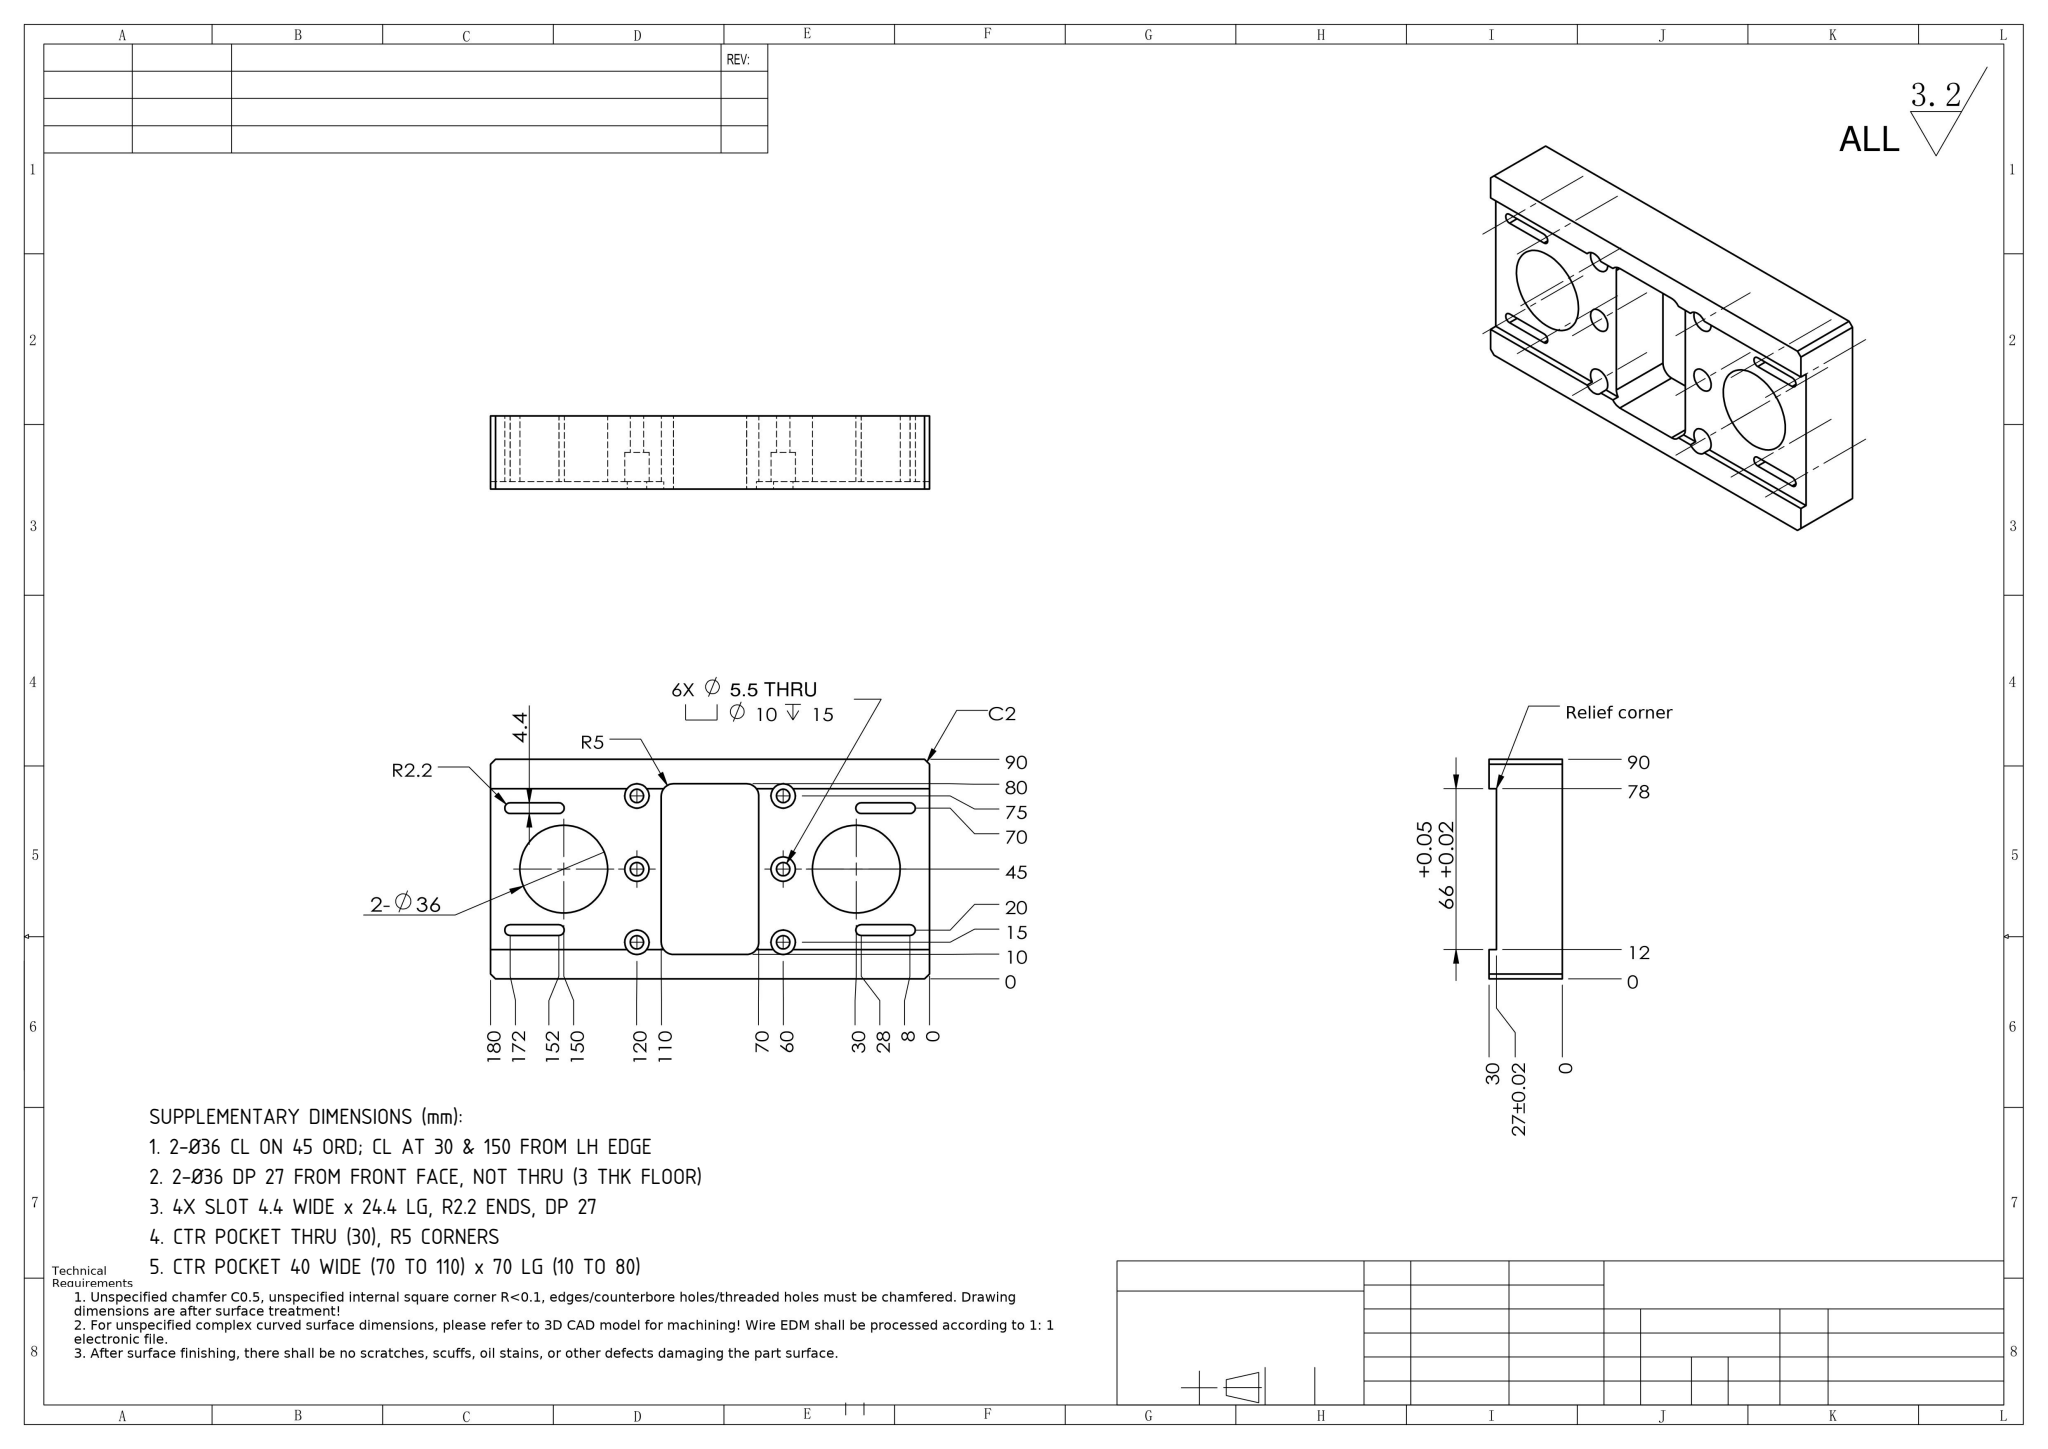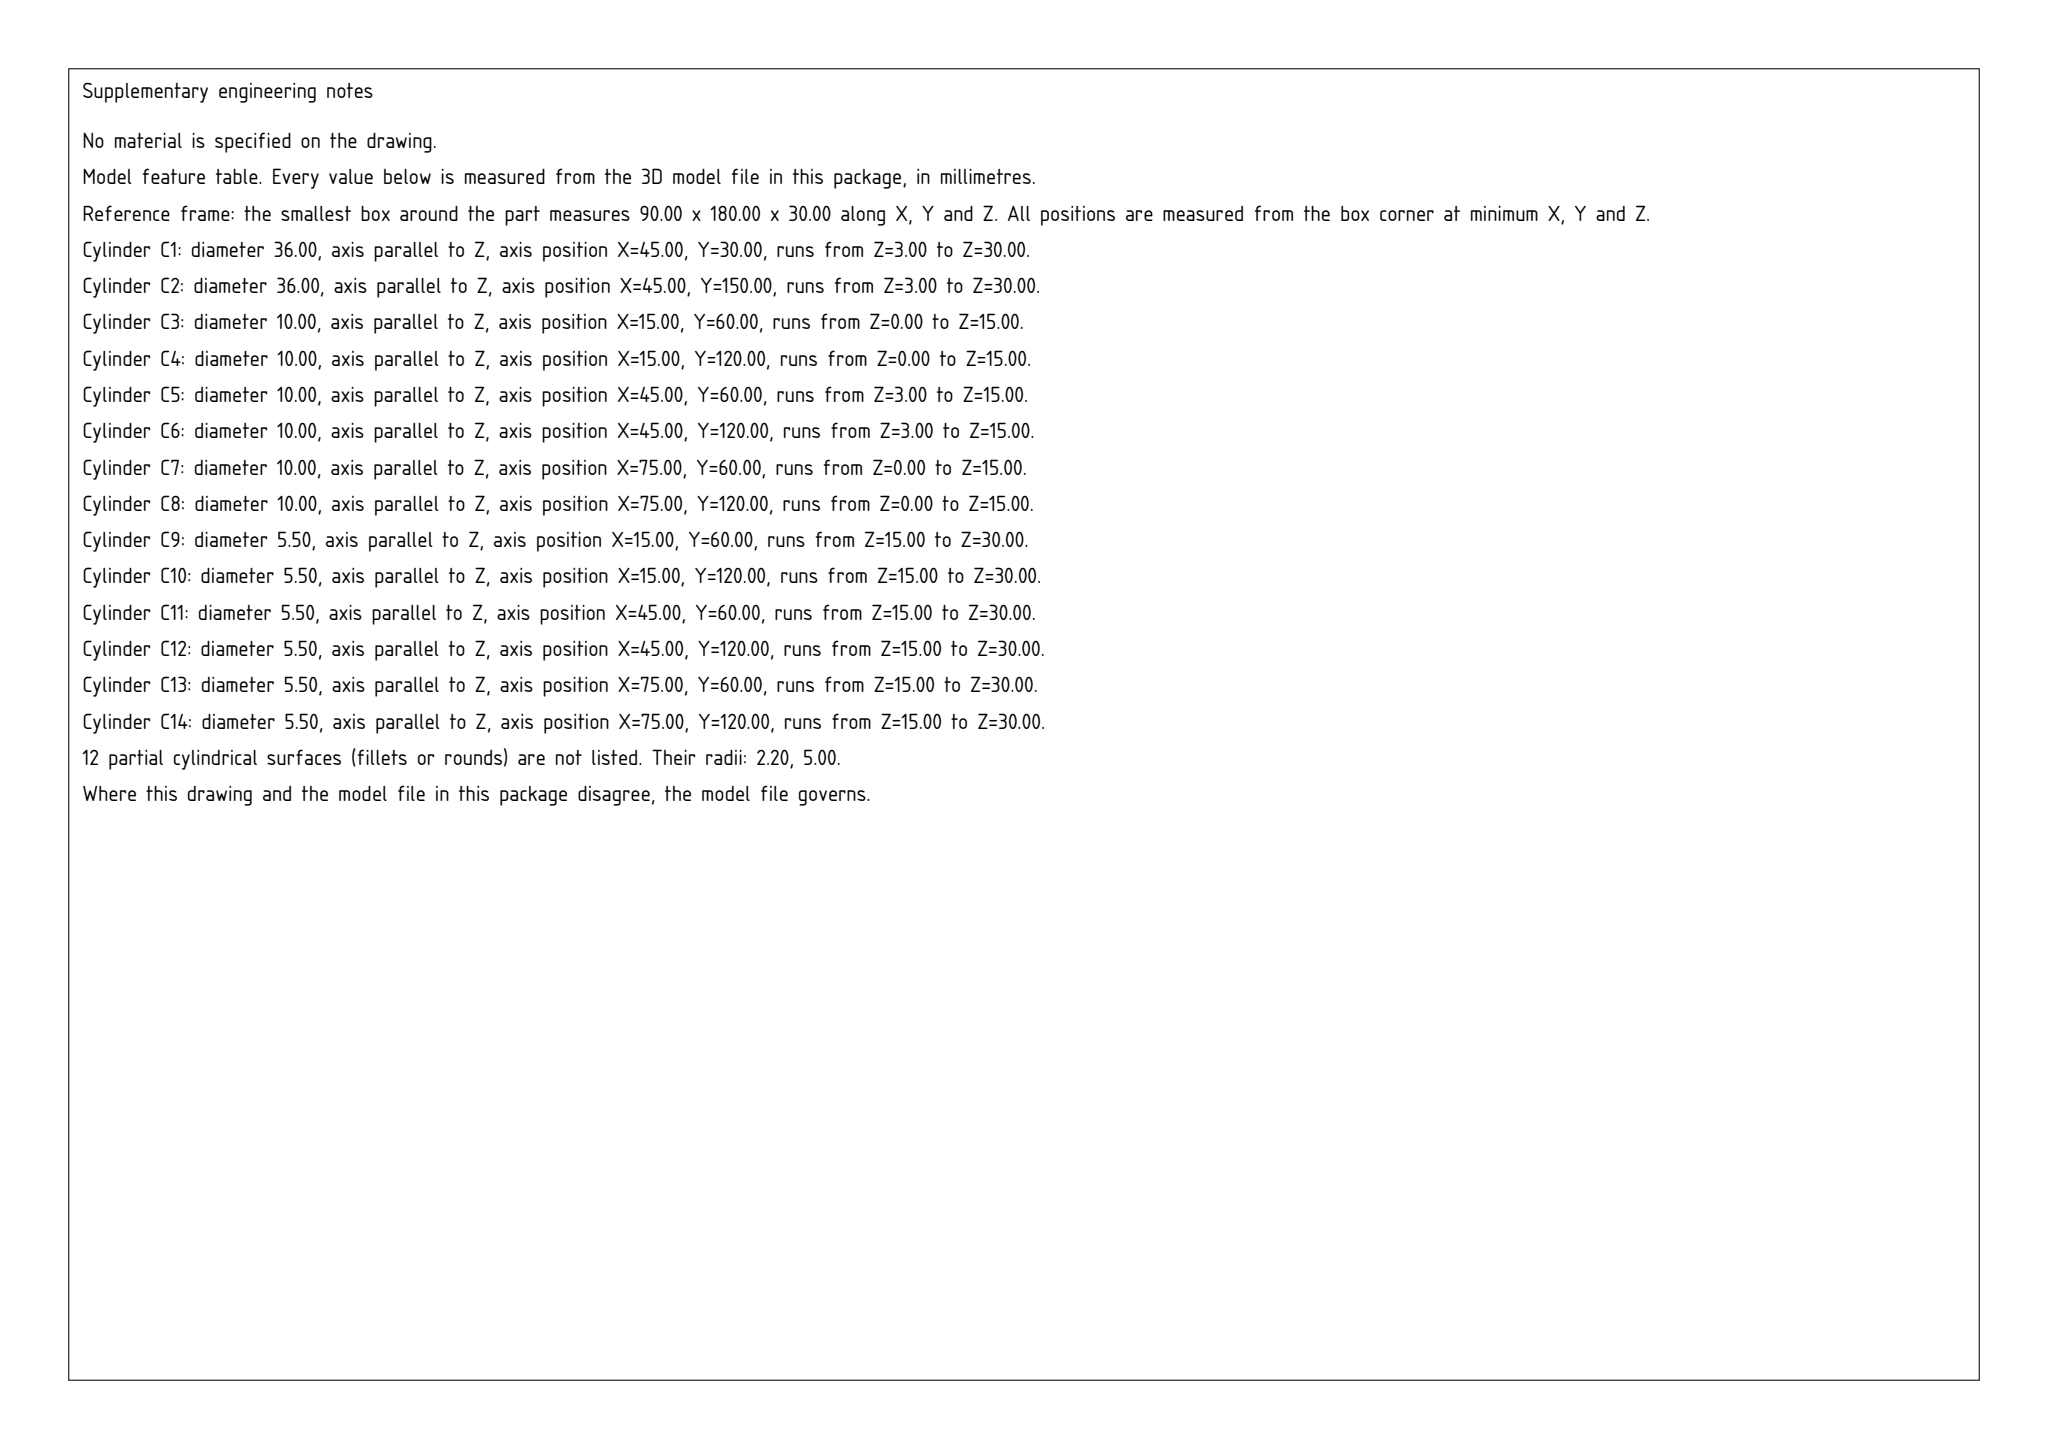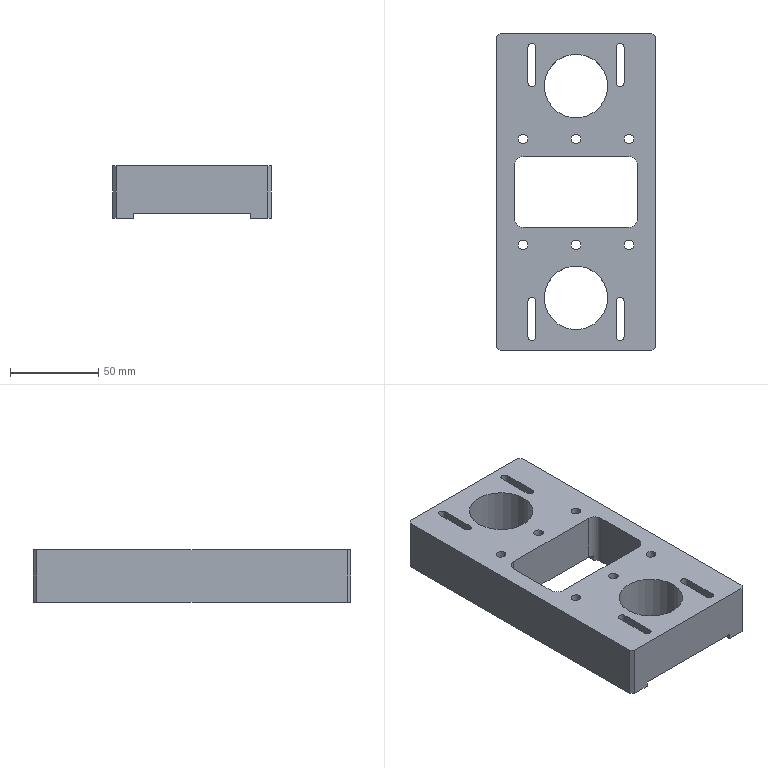Part | SolidWorks | mm | 1 solid | 79 faces | box 90 x 180 x 30 mm | volume 300634 mm3 | cylinder 40 | plane 39 | commonest cylinder face diameters 10 x16 5.5 x12 4.4 x8 36 x4
build123d program:
from build123d import *

# Parameters (mm, degrees)
SKETCH1_W                                       = 90
SKETCH1_H                                       = 180
BOSS_EXTRUDE1_DEPTH                             = 30
SKETCH2_W                                       = 66
SKETCH2_H                                       = 3
CUT_EXTRUDE1_DEPTH                              = 204.47
M5_HEX_SOCKET_HEAD_CAP_SCREW_CBORE1_D           = 5.5
M5_HEX_SOCKET_HEAD_CAP_SCREW_CBORE1_CBORE_D     = 10
M5_HEX_SOCKET_HEAD_CAP_SCREW_CBORE1_CBORE_DEPTH = 15
CUT_EXTRUDE2_DEPTH                              = 204.47
SKETCH6_R                                       = 18
SKETCH6_W                                       = 70
SKETCH6_H                                       = 40
CUT_EXTRUDE3_DEPTH                              = 204.47
FILLET1_R                                       = 5
CHAMFER1_SIZE                                   = 2


with BuildPart() as part:
    # Sketch1 → Boss-Extrude1 (new body)
    with BuildSketch(Plane.XY):
        with Locations((45, 90)):
            Rectangle(SKETCH1_W, SKETCH1_H)
    extrude(amount=BOSS_EXTRUDE1_DEPTH)

    # Sketch2 → Cut-Extrude1 (cut, through all)
    with BuildSketch(Plane(origin=(0, 180, 0), x_dir=(1, 0, 0), z_dir=(0, 1, 0))):
        with Locations((45, -1.5)):
            Rectangle(SKETCH2_W, SKETCH2_H)
    extrude(amount=-CUT_EXTRUDE1_DEPTH, mode=Mode.SUBTRACT)

    # M5 Hex Socket Head Cap Screw CBORE1 (through all)
    with Locations(Plane(origin=(0, 0, 0), x_dir=(-1, 0, 0), z_dir=(0, 0, -1))):
        with Locations((-75, 120), (-45, 120), (-15, 120), (-15, 60), (-45, 60), (-75, 60)):
            CounterBoreHole(M5_HEX_SOCKET_HEAD_CAP_SCREW_CBORE1_D / 2, M5_HEX_SOCKET_HEAD_CAP_SCREW_CBORE1_CBORE_D / 2, M5_HEX_SOCKET_HEAD_CAP_SCREW_CBORE1_CBORE_DEPTH)

    # Sketch5 → Cut-Extrude2 (cut, through all)
    with BuildSketch(Plane.XY.offset(30)):
        with BuildLine():
            Line((22.2, 172), (22.2, 152))
            ThreePointArc((22.2, 152), (20, 149.8), (17.8, 152))
            Line((17.8, 152), (17.8, 172))
            ThreePointArc((17.8, 172), (20, 174.2), (22.2, 172))
        make_face()
        with BuildLine():
            Line((72.2, 172), (72.2, 152))
            ThreePointArc((72.2, 152), (70, 149.8), (67.8, 152))
            Line((67.8, 152), (67.8, 172))
            ThreePointArc((67.8, 172), (70, 174.2), (72.2, 172))
        make_face()
        with BuildLine():
            Line((22.2, 28), (22.2, 8))
            ThreePointArc((22.2, 8), (20, 5.8), (17.8, 8))
            Line((17.8, 8), (17.8, 28))
            ThreePointArc((17.8, 28), (20, 30.2), (22.2, 28))
        make_face()
        with BuildLine():
            Line((72.2, 28), (72.2, 8))
            ThreePointArc((72.2, 8), (70, 5.8), (67.8, 8))
            Line((67.8, 8), (67.8, 28))
            ThreePointArc((67.8, 28), (70, 30.2), (72.2, 28))
        make_face()
    extrude(amount=-CUT_EXTRUDE2_DEPTH, mode=Mode.SUBTRACT)

    # Sketch6 → Cut-Extrude3 (cut, through all)
    with BuildSketch(Plane.XY.offset(30)):
        with Locations((45, 30)):
            Circle(SKETCH6_R)
        with Locations((45, 150)):
            Circle(SKETCH6_R)
        with Locations((45, 90)):
            Rectangle(SKETCH6_W, SKETCH6_H)
    extrude(amount=-CUT_EXTRUDE3_DEPTH, mode=Mode.SUBTRACT)

    # Fillet1
    fillet1_edges = [part.edges().sort_by_distance(p)[0] for p in [
        (10, 70, 15),
        (80, 70, 15),
        (80, 110, 15),
        (10, 110, 15),
    ]]
    fillet(fillet1_edges, radius=FILLET1_R)

    # Chamfer1
    chamfer1_edges = [part.edges().sort_by_distance(p)[0] for p in [
        (0, 180, 15),
        (90, 180, 15),
        (90, 0, 15),
        (0, 0, 15),
    ]]
    chamfer(chamfer1_edges, length=CHAMFER1_SIZE)


solid = part.part